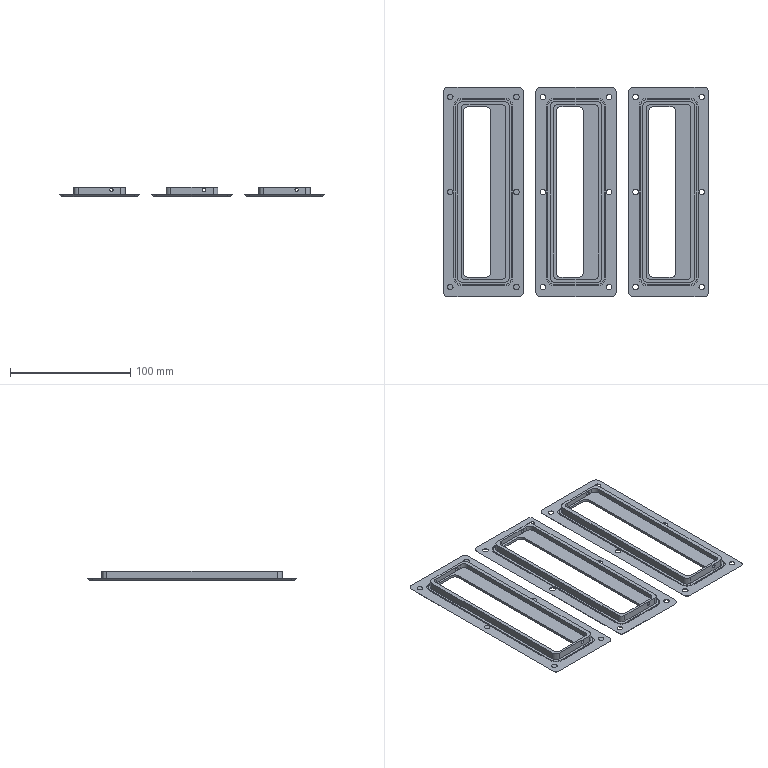CAM job | Mastercam | mm | 16 operations | part box 221 x 174 x 8
1. 3D High Speed (Area roughing) | 9 - 10 平铣刀
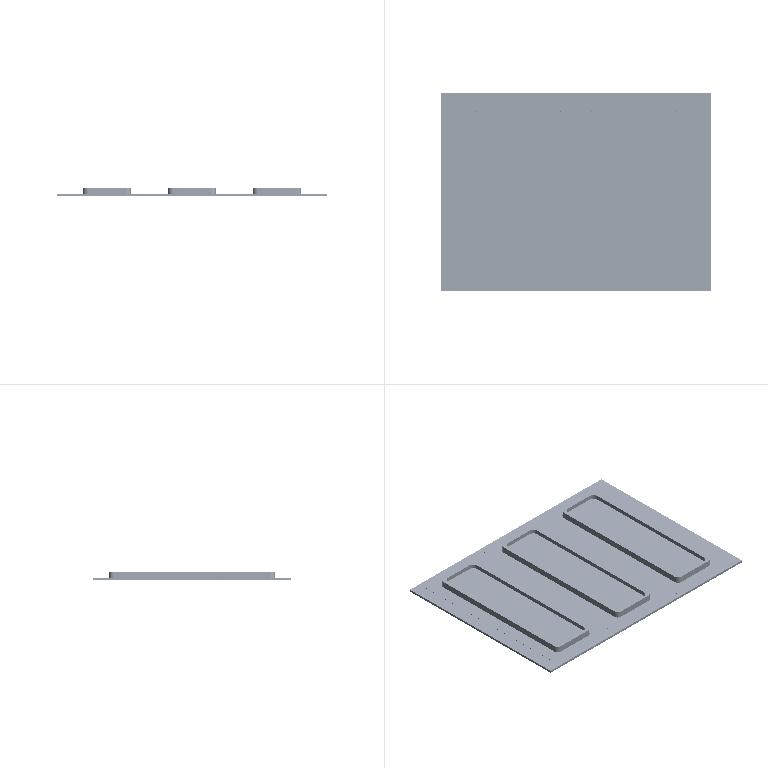2. Contour (2D) | 10 - 10 平铣刀
3. Contour (Remachining) | 8 - 8 平铣刀
4. 2D High Speed (2D Area Mill) | 8 - 8 平铣刀
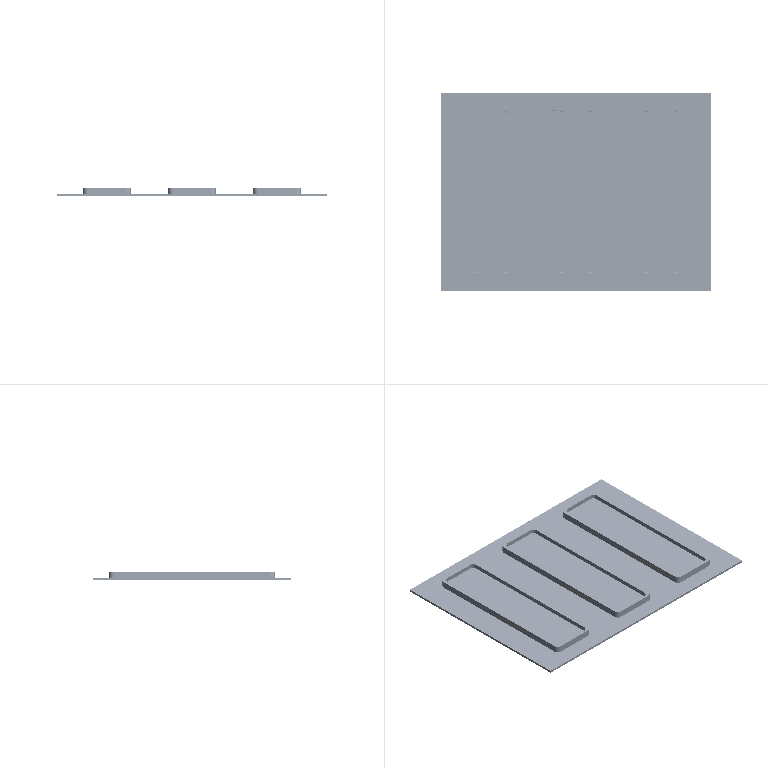5. Contour (2D) | 8 - 8 平铣刀
6. Contour (Ramp) | 1 - 1 平铣刀
7. Contour (Ramp) | 4 - 4 平铣刀
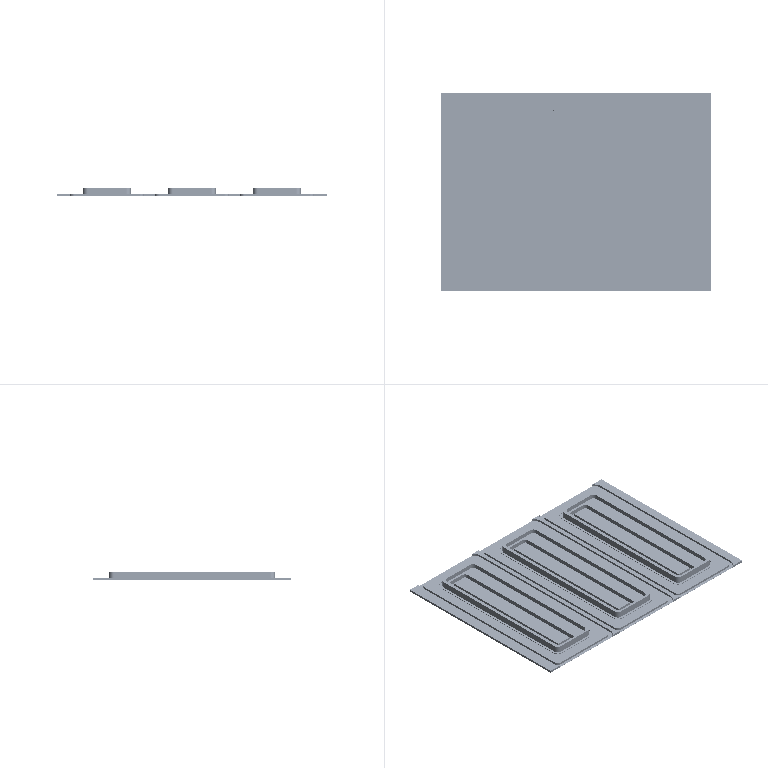8. Contour (2D chamfer) | 5 - 4 倒角刀
9. Contour (2D chamfer) | 5 - 4 倒角刀
10. Contour (2D chamfer) | 5 - 4 倒角刀
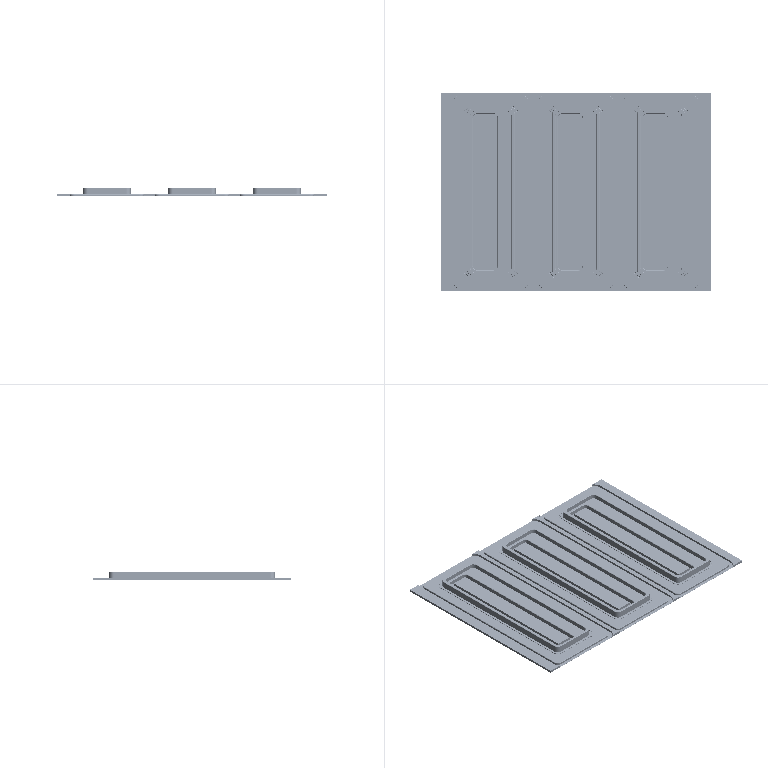11. Drill/Counterbore | 5 - 4 倒角刀
12. Contour (Ramp) | 3 - 3 平铣刀
13. Surface Finish Flowline | 14 - 4 圆鼻铣刀
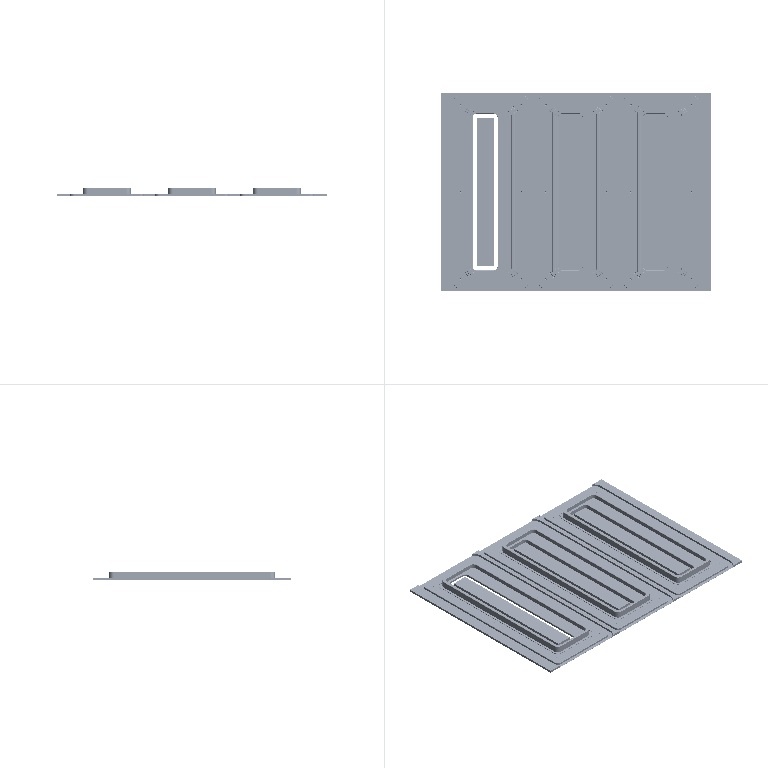14. Surface Finish Flowline | 14 - 4 圆鼻铣刀
15. Drill/Counterbore | 5 - 4 倒角刀
16. Drill/Counterbore | 5 - 4 倒角刀